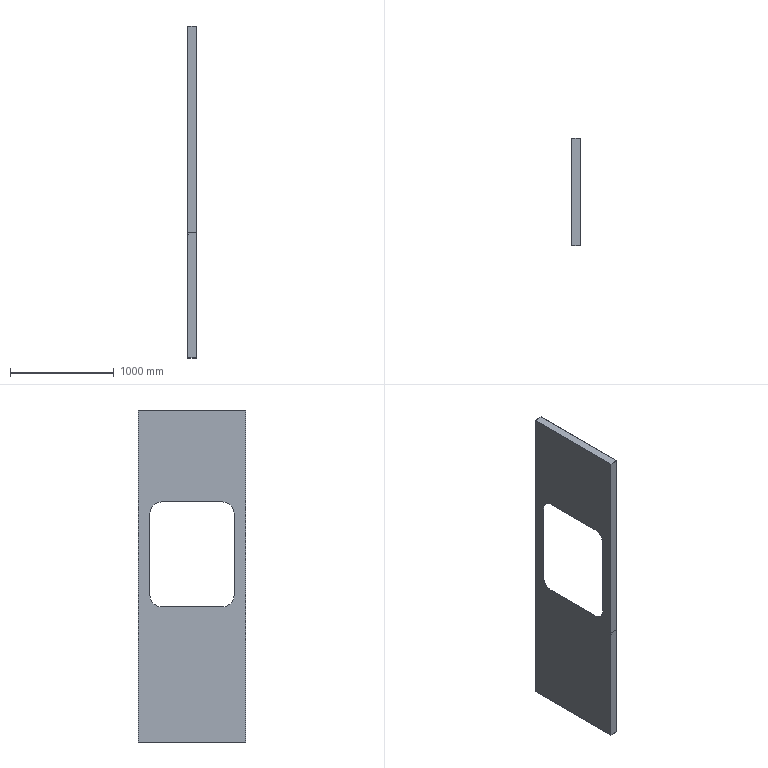Component | NX | CB2 | 1 solid | 38 faces | volume 4870461 mm3 | plane 34 | cylinder 4 | commonest cylinder face diameters 218 x4